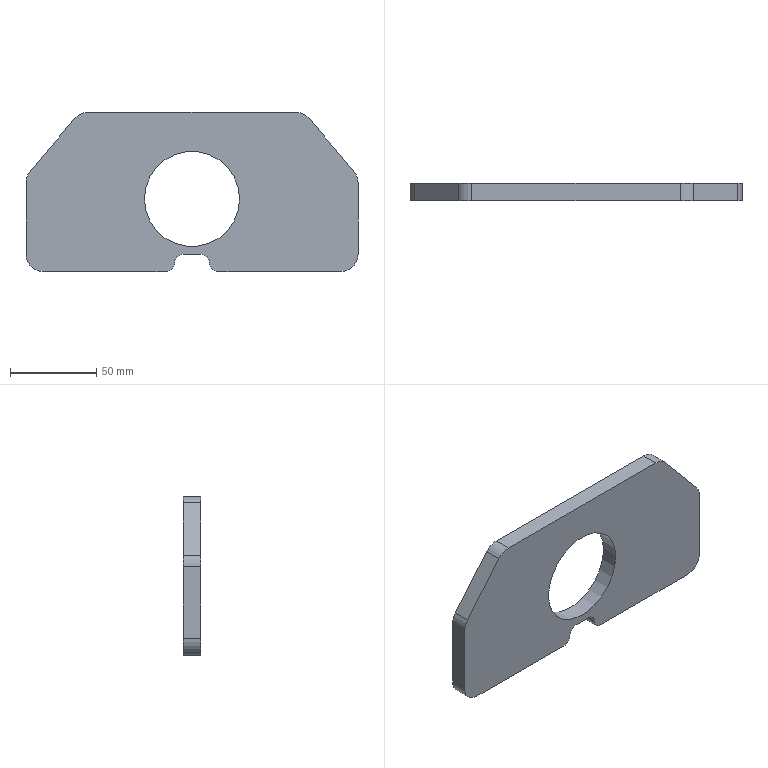Component | SolidWorks | HangingChannelAssembly-2_LiftingLug-3 | 1 solid | 22 faces | box 192 x 10 x 92 mm | volume 138893 mm3 | cylinder 12 | plane 10 | commonest cylinder face diameters 20 x6 10 x4 55 x2 | material Plain Carbon Steel
STEP:
#1=COLOUR_RGB('',0.7922,0.8196,0.9333);
#2=FILL_AREA_STYLE_COLOUR('',#1);
#3=FILL_AREA_STYLE('',(#2));
#4=SURFACE_STYLE_FILL_AREA(#3);
#5=SURFACE_SIDE_STYLE('',(#4));
#6=SURFACE_STYLE_USAGE(.BOTH.,#5);
#7=PRESENTATION_STYLE_ASSIGNMENT((#6));
#8=CARTESIAN_POINT('',(18.377,47.62,81.554));
#9=VERTEX_POINT('',#8);
#10=CARTESIAN_POINT('',(16.212,47.62,81.554));
#11=VERTEX_POINT('',#10);
#12=CARTESIAN_POINT('',(17.295,47.62,81.554));
#13=DIRECTION('',(0.,1.,-0.));
#14=DIRECTION('',(-1.,0.,0.));
#15=AXIS2_PLACEMENT_3D('',#12,#13,#14);
#16=CIRCLE('',#15,1.083);
#17=EDGE_CURVE('',#9,#11,#16,.T.);
#18=ORIENTED_EDGE('',*,*,#17,.T.);
#19=CARTESIAN_POINT('',(16.212,47.226,81.554));
#20=VERTEX_POINT('',#19);
#21=CARTESIAN_POINT('',(16.212,47.62,81.554));
#22=DIRECTION('',(-0.,-1.,0.));
#23=VECTOR('',#22,39.37);
#24=LINE('',#21,#23);
#25=EDGE_CURVE('',#11,#20,#24,.T.);
#26=ORIENTED_EDGE('',*,*,#25,.T.);
#27=CARTESIAN_POINT('',(18.377,47.226,81.554));
#28=VERTEX_POINT('',#27);
#29=CARTESIAN_POINT('',(17.295,47.226,81.554));
#30=DIRECTION('',(0.,1.,-0.));
#31=DIRECTION('',(-1.,0.,0.));
#32=AXIS2_PLACEMENT_3D('',#29,#30,#31);
#33=CIRCLE('',#32,1.083);
#34=EDGE_CURVE('',#28,#20,#33,.T.);
#35=ORIENTED_EDGE('',*,*,#34,.F.);
#36=CARTESIAN_POINT('',(18.377,47.62,81.554));
#37=DIRECTION('',(-0.,-1.,0.));
#38=VECTOR('',#37,39.37);
#39=LINE('',#36,#38);
#40=EDGE_CURVE('',#9,#28,#39,.T.);
#41=ORIENTED_EDGE('',*,*,#40,.F.);
#42=EDGE_LOOP('',(#18,#26,#35,#41));
#43=FACE_OUTER_BOUND('',#42,.T.);
#44=CARTESIAN_POINT('',(17.295,47.62,81.554));
#45=DIRECTION('',(-0.,-1.,0.));
#46=DIRECTION('',(1.,0.,0.));
#47=AXIS2_PLACEMENT_3D('',#44,#45,#46);
#48=CYLINDRICAL_SURFACE('',#47,1.083);
#49=ADVANCED_FACE('',(#43),#48,.F.);
#50=CARTESIAN_POINT('',(16.704,47.62,79.901));
#51=VERTEX_POINT('',#50);
#52=CARTESIAN_POINT('',(13.909,47.62,79.901));
#53=VERTEX_POINT('',#52);
#54=CARTESIAN_POINT('',(21.074,47.62,79.901));
#55=DIRECTION('',(-1.,0.,-0.));
#56=VECTOR('',#55,39.37);
#57=LINE('',#54,#56);
#58=EDGE_CURVE('',#51,#53,#57,.T.);
#59=ORIENTED_EDGE('',*,*,#58,.F.);
#60=CARTESIAN_POINT('',(16.704,47.226,79.901));
#61=VERTEX_POINT('',#60);
#62=CARTESIAN_POINT('',(16.704,47.62,79.901));
#63=DIRECTION('',(-0.,-1.,0.));
#64=VECTOR('',#63,39.37);
#65=LINE('',#62,#64);
#66=EDGE_CURVE('',#51,#61,#65,.T.);
#67=ORIENTED_EDGE('',*,*,#66,.T.);
#68=CARTESIAN_POINT('',(13.909,47.226,79.901));
#69=VERTEX_POINT('',#68);
#70=CARTESIAN_POINT('',(21.074,47.226,79.901));
#71=DIRECTION('',(-1.,0.,-0.));
#72=VECTOR('',#71,39.37);
#73=LINE('',#70,#72);
#74=EDGE_CURVE('',#61,#69,#73,.T.);
#75=ORIENTED_EDGE('',*,*,#74,.T.);
#76=CARTESIAN_POINT('',(13.909,47.62,79.901));
#77=DIRECTION('',(0.,1.,-0.));
#78=VECTOR('',#77,39.37);
#79=LINE('',#76,#78);
#80=EDGE_CURVE('',#69,#53,#79,.T.);
#81=ORIENTED_EDGE('',*,*,#80,.T.);
#82=EDGE_LOOP('',(#59,#67,#75,#81));
#83=FACE_OUTER_BOUND('',#82,.T.);
#84=CARTESIAN_POINT('',(21.074,47.62,79.901));
#85=DIRECTION('',(0.,0.,1.));
#86=DIRECTION('',(0.,1.,-0.));
#87=AXIS2_PLACEMENT_3D('',#84,#85,#86);
#88=PLANE('',#87);
#89=ADVANCED_FACE('',(#83),#88,.F.);
#90=CARTESIAN_POINT('',(17.492,47.62,80.294));
#91=VERTEX_POINT('',#90);
#92=CARTESIAN_POINT('',(17.098,47.62,80.294));
#93=VERTEX_POINT('',#92);
#94=CARTESIAN_POINT('',(16.901,47.62,80.294));
#95=DIRECTION('',(-1.,0.,-0.));
#96=VECTOR('',#95,39.37);
#97=LINE('',#94,#96);
#98=EDGE_CURVE('',#91,#93,#97,.T.);
#99=ORIENTED_EDGE('',*,*,#98,.T.);
#100=CARTESIAN_POINT('',(16.901,47.62,80.098));
#101=VERTEX_POINT('',#100);
#102=CARTESIAN_POINT('',(17.098,47.62,80.098));
#103=DIRECTION('',(-0.,-1.,0.));
#104=DIRECTION('',(-1.,0.,0.));
#105=AXIS2_PLACEMENT_3D('',#102,#103,#104);
#106=CIRCLE('',#105,0.1969);
#107=EDGE_CURVE('',#93,#101,#106,.T.);
#108=ORIENTED_EDGE('',*,*,#107,.T.);
#109=CARTESIAN_POINT('',(16.704,47.62,80.098));
#110=DIRECTION('',(0.,1.,-0.));
#111=DIRECTION('',(-1.,0.,0.));
#112=AXIS2_PLACEMENT_3D('',#109,#110,#111);
#113=CIRCLE('',#112,0.1969);
#114=EDGE_CURVE('',#101,#51,#113,.T.);
#115=ORIENTED_EDGE('',*,*,#114,.T.);
#116=ORIENTED_EDGE('',*,*,#58,.T.);
#117=CARTESIAN_POINT('',(13.515,47.62,80.294));
#118=VERTEX_POINT('',#117);
#119=CARTESIAN_POINT('',(13.909,47.62,80.294));
#120=DIRECTION('',(0.,1.,-0.));
#121=DIRECTION('',(-1.,0.,0.));
#122=AXIS2_PLACEMENT_3D('',#119,#120,#121);
#123=CIRCLE('',#122,0.3937);
#124=EDGE_CURVE('',#53,#118,#123,.T.);
#125=ORIENTED_EDGE('',*,*,#124,.T.);
#126=CARTESIAN_POINT('',(13.515,47.62,81.923));
#127=VERTEX_POINT('',#126);
#128=CARTESIAN_POINT('',(13.515,47.62,79.901));
#129=DIRECTION('',(0.,0.,1.));
#130=VECTOR('',#129,39.37);
#131=LINE('',#128,#130);
#132=EDGE_CURVE('',#118,#127,#131,.T.);
#133=ORIENTED_EDGE('',*,*,#132,.T.);
#134=CARTESIAN_POINT('',(13.607,47.62,82.176));
#135=VERTEX_POINT('',#134);
#136=CARTESIAN_POINT('',(13.909,47.62,81.923));
#137=DIRECTION('',(0.,1.,-0.));
#138=DIRECTION('',(-1.,0.,0.));
#139=AXIS2_PLACEMENT_3D('',#136,#137,#138);
#140=CIRCLE('',#139,0.3937);
#141=EDGE_CURVE('',#127,#135,#140,.T.);
#142=ORIENTED_EDGE('',*,*,#141,.T.);
#143=CARTESIAN_POINT('',(14.618,47.62,83.382));
#144=VERTEX_POINT('',#143);
#145=CARTESIAN_POINT('',(14.736,47.62,83.523));
#146=DIRECTION('',(0.6422,0.,0.7665));
#147=VECTOR('',#146,39.37);
#148=LINE('',#145,#147);
#149=EDGE_CURVE('',#135,#144,#148,.T.);
#150=ORIENTED_EDGE('',*,*,#149,.T.);
#151=CARTESIAN_POINT('',(14.919,47.62,83.523));
#152=VERTEX_POINT('',#151);
#153=CARTESIAN_POINT('',(14.919,47.62,83.129));
#154=DIRECTION('',(0.,1.,-0.));
#155=DIRECTION('',(-1.,0.,0.));
#156=AXIS2_PLACEMENT_3D('',#153,#154,#155);
#157=CIRCLE('',#156,0.3937);
#158=EDGE_CURVE('',#144,#152,#157,.T.);
#159=ORIENTED_EDGE('',*,*,#158,.T.);
#160=CARTESIAN_POINT('',(19.67,47.62,83.523));
#161=VERTEX_POINT('',#160);
#162=CARTESIAN_POINT('',(14.736,47.62,83.523));
#163=DIRECTION('',(1.,-0.,-0.));
#164=VECTOR('',#163,39.37);
#165=LINE('',#162,#164);
#166=EDGE_CURVE('',#152,#161,#165,.T.);
#167=ORIENTED_EDGE('',*,*,#166,.T.);
#168=CARTESIAN_POINT('',(19.972,47.62,83.382));
#169=VERTEX_POINT('',#168);
#170=CARTESIAN_POINT('',(19.67,47.62,83.129));
#171=DIRECTION('',(0.,1.,-0.));
#172=DIRECTION('',(-1.,0.,0.));
#173=AXIS2_PLACEMENT_3D('',#170,#171,#172);
#174=CIRCLE('',#173,0.3937);
#175=EDGE_CURVE('',#161,#169,#174,.T.);
#176=ORIENTED_EDGE('',*,*,#175,.T.);
#177=CARTESIAN_POINT('',(20.982,47.62,82.176));
#178=VERTEX_POINT('',#177);
#179=CARTESIAN_POINT('',(19.854,47.62,83.523));
#180=DIRECTION('',(0.6422,-0.,-0.7665));
#181=VECTOR('',#180,39.37);
#182=LINE('',#179,#181);
#183=EDGE_CURVE('',#169,#178,#182,.T.);
#184=ORIENTED_EDGE('',*,*,#183,.T.);
#185=CARTESIAN_POINT('',(21.074,47.62,81.923));
#186=VERTEX_POINT('',#185);
#187=CARTESIAN_POINT('',(20.681,47.62,81.923));
#188=DIRECTION('',(0.,1.,-0.));
#189=DIRECTION('',(-1.,0.,0.));
#190=AXIS2_PLACEMENT_3D('',#187,#188,#189);
#191=CIRCLE('',#190,0.3937);
#192=EDGE_CURVE('',#178,#186,#191,.T.);
#193=ORIENTED_EDGE('',*,*,#192,.T.);
#194=CARTESIAN_POINT('',(21.074,47.62,80.294));
#195=VERTEX_POINT('',#194);
#196=CARTESIAN_POINT('',(21.074,47.62,79.901));
#197=DIRECTION('',(-0.,-0.,-1.));
#198=VECTOR('',#197,39.37);
#199=LINE('',#196,#198);
#200=EDGE_CURVE('',#186,#195,#199,.T.);
#201=ORIENTED_EDGE('',*,*,#200,.T.);
#202=CARTESIAN_POINT('',(20.681,47.62,79.901));
#203=VERTEX_POINT('',#202);
#204=CARTESIAN_POINT('',(20.681,47.62,80.294));
#205=DIRECTION('',(0.,1.,-0.));
#206=DIRECTION('',(-1.,0.,0.));
#207=AXIS2_PLACEMENT_3D('',#204,#205,#206);
#208=CIRCLE('',#207,0.3937);
#209=EDGE_CURVE('',#195,#203,#208,.T.);
#210=ORIENTED_EDGE('',*,*,#209,.T.);
#211=CARTESIAN_POINT('',(17.885,47.62,79.901));
#212=VERTEX_POINT('',#211);
#213=CARTESIAN_POINT('',(21.074,47.62,79.901));
#214=DIRECTION('',(-1.,0.,-0.));
#215=VECTOR('',#214,39.37);
#216=LINE('',#213,#215);
#217=EDGE_CURVE('',#203,#212,#216,.T.);
#218=ORIENTED_EDGE('',*,*,#217,.T.);
#219=CARTESIAN_POINT('',(17.688,47.62,80.098));
#220=VERTEX_POINT('',#219);
#221=CARTESIAN_POINT('',(17.885,47.62,80.098));
#222=DIRECTION('',(0.,1.,-0.));
#223=DIRECTION('',(-1.,0.,0.));
#224=AXIS2_PLACEMENT_3D('',#221,#222,#223);
#225=CIRCLE('',#224,0.1969);
#226=EDGE_CURVE('',#212,#220,#225,.T.);
#227=ORIENTED_EDGE('',*,*,#226,.T.);
#228=CARTESIAN_POINT('',(17.492,47.62,80.098));
#229=DIRECTION('',(-0.,-1.,0.));
#230=DIRECTION('',(-1.,0.,0.));
#231=AXIS2_PLACEMENT_3D('',#228,#229,#230);
#232=CIRCLE('',#231,0.1969);
#233=EDGE_CURVE('',#220,#91,#232,.T.);
#234=ORIENTED_EDGE('',*,*,#233,.T.);
#235=EDGE_LOOP('',(#99,#108,#115,#116,#125,#133,#142,#150,#159,#167,#176,#184,#193,#201,#210,#218,#227,#234));
#236=FACE_OUTER_BOUND('',#235,.T.);
#237=ORIENTED_EDGE('',*,*,#17,.F.);
#238=CARTESIAN_POINT('',(17.295,47.62,81.554));
#239=DIRECTION('',(0.,1.,-0.));
#240=DIRECTION('',(-1.,0.,0.));
#241=AXIS2_PLACEMENT_3D('',#238,#239,#240);
#242=CIRCLE('',#241,1.083);
#243=EDGE_CURVE('',#11,#9,#242,.T.);
#244=ORIENTED_EDGE('',*,*,#243,.F.);
#245=EDGE_LOOP('',(#237,#244));
#246=FACE_BOUND('',#245,.T.);
#247=CARTESIAN_POINT('',(21.074,47.62,79.901));
#248=DIRECTION('',(0.,1.,-0.));
#249=DIRECTION('',(-1.,0.,-0.));
#250=AXIS2_PLACEMENT_3D('',#247,#248,#249);
#251=PLANE('',#250);
#252=ADVANCED_FACE('',(#236,#246),#251,.T.);
#253=ORIENTED_EDGE('',*,*,#74,.F.);
#254=CARTESIAN_POINT('',(16.901,47.226,80.098));
#255=VERTEX_POINT('',#254);
#256=CARTESIAN_POINT('',(16.704,47.226,80.098));
#257=DIRECTION('',(-0.,-1.,0.));
#258=DIRECTION('',(-1.,0.,0.));
#259=AXIS2_PLACEMENT_3D('',#256,#257,#258);
#260=CIRCLE('',#259,0.1969);
#261=EDGE_CURVE('',#61,#255,#260,.T.);
#262=ORIENTED_EDGE('',*,*,#261,.T.);
#263=CARTESIAN_POINT('',(17.098,47.226,80.294));
#264=VERTEX_POINT('',#263);
#265=CARTESIAN_POINT('',(17.098,47.226,80.098));
#266=DIRECTION('',(0.,1.,-0.));
#267=DIRECTION('',(-1.,0.,0.));
#268=AXIS2_PLACEMENT_3D('',#265,#266,#267);
#269=CIRCLE('',#268,0.1969);
#270=EDGE_CURVE('',#255,#264,#269,.T.);
#271=ORIENTED_EDGE('',*,*,#270,.T.);
#272=CARTESIAN_POINT('',(17.492,47.226,80.294));
#273=VERTEX_POINT('',#272);
#274=CARTESIAN_POINT('',(16.901,47.226,80.294));
#275=DIRECTION('',(-1.,0.,-0.));
#276=VECTOR('',#275,39.37);
#277=LINE('',#274,#276);
#278=EDGE_CURVE('',#273,#264,#277,.T.);
#279=ORIENTED_EDGE('',*,*,#278,.F.);
#280=CARTESIAN_POINT('',(17.688,47.226,80.098));
#281=VERTEX_POINT('',#280);
#282=CARTESIAN_POINT('',(17.492,47.226,80.098));
#283=DIRECTION('',(0.,1.,-0.));
#284=DIRECTION('',(-1.,0.,0.));
#285=AXIS2_PLACEMENT_3D('',#282,#283,#284);
#286=CIRCLE('',#285,0.1969);
#287=EDGE_CURVE('',#273,#281,#286,.T.);
#288=ORIENTED_EDGE('',*,*,#287,.T.);
#289=CARTESIAN_POINT('',(17.885,47.226,79.901));
#290=VERTEX_POINT('',#289);
#291=CARTESIAN_POINT('',(17.885,47.226,80.098));
#292=DIRECTION('',(-0.,-1.,0.));
#293=DIRECTION('',(-1.,0.,0.));
#294=AXIS2_PLACEMENT_3D('',#291,#292,#293);
#295=CIRCLE('',#294,0.1969);
#296=EDGE_CURVE('',#281,#290,#295,.T.);
#297=ORIENTED_EDGE('',*,*,#296,.T.);
#298=CARTESIAN_POINT('',(20.681,47.226,79.901));
#299=VERTEX_POINT('',#298);
#300=CARTESIAN_POINT('',(21.074,47.226,79.901));
#301=DIRECTION('',(-1.,0.,-0.));
#302=VECTOR('',#301,39.37);
#303=LINE('',#300,#302);
#304=EDGE_CURVE('',#299,#290,#303,.T.);
#305=ORIENTED_EDGE('',*,*,#304,.F.);
#306=CARTESIAN_POINT('',(21.074,47.226,80.294));
#307=VERTEX_POINT('',#306);
#308=CARTESIAN_POINT('',(20.681,47.226,80.294));
#309=DIRECTION('',(-0.,-1.,0.));
#310=DIRECTION('',(-1.,0.,0.));
#311=AXIS2_PLACEMENT_3D('',#308,#309,#310);
#312=CIRCLE('',#311,0.3937);
#313=EDGE_CURVE('',#299,#307,#312,.T.);
#314=ORIENTED_EDGE('',*,*,#313,.T.);
#315=CARTESIAN_POINT('',(21.074,47.226,81.923));
#316=VERTEX_POINT('',#315);
#317=CARTESIAN_POINT('',(21.074,47.226,79.901));
#318=DIRECTION('',(-0.,-0.,-1.));
#319=VECTOR('',#318,39.37);
#320=LINE('',#317,#319);
#321=EDGE_CURVE('',#316,#307,#320,.T.);
#322=ORIENTED_EDGE('',*,*,#321,.F.);
#323=CARTESIAN_POINT('',(20.982,47.226,82.176));
#324=VERTEX_POINT('',#323);
#325=CARTESIAN_POINT('',(20.681,47.226,81.923));
#326=DIRECTION('',(-0.,-1.,0.));
#327=DIRECTION('',(-1.,0.,-0.));
#328=AXIS2_PLACEMENT_3D('',#325,#326,#327);
#329=CIRCLE('',#328,0.3937);
#330=EDGE_CURVE('',#316,#324,#329,.T.);
#331=ORIENTED_EDGE('',*,*,#330,.T.);
#332=CARTESIAN_POINT('',(19.972,47.226,83.382));
#333=VERTEX_POINT('',#332);
#334=CARTESIAN_POINT('',(19.854,47.226,83.523));
#335=DIRECTION('',(0.6422,-0.,-0.7665));
#336=VECTOR('',#335,39.37);
#337=LINE('',#334,#336);
#338=EDGE_CURVE('',#333,#324,#337,.T.);
#339=ORIENTED_EDGE('',*,*,#338,.F.);
#340=CARTESIAN_POINT('',(19.67,47.226,83.523));
#341=VERTEX_POINT('',#340);
#342=CARTESIAN_POINT('',(19.67,47.226,83.129));
#343=DIRECTION('',(-0.,-1.,0.));
#344=DIRECTION('',(-1.,0.,0.));
#345=AXIS2_PLACEMENT_3D('',#342,#343,#344);
#346=CIRCLE('',#345,0.3937);
#347=EDGE_CURVE('',#333,#341,#346,.T.);
#348=ORIENTED_EDGE('',*,*,#347,.T.);
#349=CARTESIAN_POINT('',(14.919,47.226,83.523));
#350=VERTEX_POINT('',#349);
#351=CARTESIAN_POINT('',(14.736,47.226,83.523));
#352=DIRECTION('',(1.,-0.,-0.));
#353=VECTOR('',#352,39.37);
#354=LINE('',#351,#353);
#355=EDGE_CURVE('',#350,#341,#354,.T.);
#356=ORIENTED_EDGE('',*,*,#355,.F.);
#357=CARTESIAN_POINT('',(14.618,47.226,83.382));
#358=VERTEX_POINT('',#357);
#359=CARTESIAN_POINT('',(14.919,47.226,83.129));
#360=DIRECTION('',(-0.,-1.,0.));
#361=DIRECTION('',(-1.,0.,0.));
#362=AXIS2_PLACEMENT_3D('',#359,#360,#361);
#363=CIRCLE('',#362,0.3937);
#364=EDGE_CURVE('',#350,#358,#363,.T.);
#365=ORIENTED_EDGE('',*,*,#364,.T.);
#366=CARTESIAN_POINT('',(13.607,47.226,82.176));
#367=VERTEX_POINT('',#366);
#368=CARTESIAN_POINT('',(14.736,47.226,83.523));
#369=DIRECTION('',(0.6422,0.,0.7665));
#370=VECTOR('',#369,39.37);
#371=LINE('',#368,#370);
#372=EDGE_CURVE('',#367,#358,#371,.T.);
#373=ORIENTED_EDGE('',*,*,#372,.F.);
#374=CARTESIAN_POINT('',(13.515,47.226,81.923));
#375=VERTEX_POINT('',#374);
#376=CARTESIAN_POINT('',(13.909,47.226,81.923));
#377=DIRECTION('',(-0.,-1.,0.));
#378=DIRECTION('',(-1.,0.,0.));
#379=AXIS2_PLACEMENT_3D('',#376,#377,#378);
#380=CIRCLE('',#379,0.3937);
#381=EDGE_CURVE('',#367,#375,#380,.T.);
#382=ORIENTED_EDGE('',*,*,#381,.T.);
#383=CARTESIAN_POINT('',(13.515,47.226,80.294));
#384=VERTEX_POINT('',#383);
#385=CARTESIAN_POINT('',(13.515,47.226,79.901));
#386=DIRECTION('',(0.,0.,1.));
#387=VECTOR('',#386,39.37);
#388=LINE('',#385,#387);
#389=EDGE_CURVE('',#384,#375,#388,.T.);
#390=ORIENTED_EDGE('',*,*,#389,.F.);
#391=CARTESIAN_POINT('',(13.909,47.226,80.294));
#392=DIRECTION('',(-0.,-1.,0.));
#393=DIRECTION('',(-1.,0.,0.));
#394=AXIS2_PLACEMENT_3D('',#391,#392,#393);
#395=CIRCLE('',#394,0.3937);
#396=EDGE_CURVE('',#384,#69,#395,.T.);
#397=ORIENTED_EDGE('',*,*,#396,.T.);
#398=EDGE_LOOP('',(#253,#262,#271,#279,#288,#297,#305,#314,#322,#331,#339,#348,#356,#365,#373,#382,#390,#397));
#399=FACE_OUTER_BOUND('',#398,.T.);
#400=ORIENTED_EDGE('',*,*,#34,.T.);
#401=CARTESIAN_POINT('',(17.295,47.226,81.554));
#402=DIRECTION('',(0.,1.,-0.));
#403=DIRECTION('',(-1.,0.,0.));
#404=AXIS2_PLACEMENT_3D('',#401,#402,#403);
#405=CIRCLE('',#404,1.083);
#406=EDGE_CURVE('',#20,#28,#405,.T.);
#407=ORIENTED_EDGE('',*,*,#406,.T.);
#408=EDGE_LOOP('',(#400,#407));
#409=FACE_BOUND('',#408,.T.);
#410=CARTESIAN_POINT('',(21.074,47.226,79.901));
#411=DIRECTION('',(0.,1.,-0.));
#412=DIRECTION('',(-1.,0.,-0.));
#413=AXIS2_PLACEMENT_3D('',#410,#411,#412);
#414=PLANE('',#413);
#415=ADVANCED_FACE('',(#399,#409),#414,.F.);
#416=ORIENTED_EDGE('',*,*,#200,.F.);
#417=CARTESIAN_POINT('',(21.074,47.62,81.923));
#418=DIRECTION('',(-0.,-1.,0.));
#419=VECTOR('',#418,39.37);
#420=LINE('',#417,#419);
#421=EDGE_CURVE('',#186,#316,#420,.T.);
#422=ORIENTED_EDGE('',*,*,#421,.T.);
#423=ORIENTED_EDGE('',*,*,#321,.T.);
#424=CARTESIAN_POINT('',(21.074,47.62,80.294));
#425=DIRECTION('',(0.,1.,-0.));
#426=VECTOR('',#425,39.37);
#427=LINE('',#424,#426);
#428=EDGE_CURVE('',#307,#195,#427,.T.);
#429=ORIENTED_EDGE('',*,*,#428,.T.);
#430=EDGE_LOOP('',(#416,#422,#423,#429));
#431=FACE_OUTER_BOUND('',#430,.T.);
#432=CARTESIAN_POINT('',(21.074,47.62,79.901));
#433=DIRECTION('',(-1.,0.,0.));
#434=DIRECTION('',(-0.,-1.,0.));
#435=AXIS2_PLACEMENT_3D('',#432,#433,#434);
#436=PLANE('',#435);
#437=ADVANCED_FACE('',(#431),#436,.F.);
#438=ORIENTED_EDGE('',*,*,#304,.T.);
#439=CARTESIAN_POINT('',(17.885,47.62,79.901));
#440=DIRECTION('',(0.,1.,-0.));
#441=VECTOR('',#440,39.37);
#442=LINE('',#439,#441);
#443=EDGE_CURVE('',#290,#212,#442,.T.);
#444=ORIENTED_EDGE('',*,*,#443,.T.);
#445=ORIENTED_EDGE('',*,*,#217,.F.);
#446=CARTESIAN_POINT('',(20.681,47.62,79.901));
#447=DIRECTION('',(-0.,-1.,0.));
#448=VECTOR('',#447,39.37);
#449=LINE('',#446,#448);
#450=EDGE_CURVE('',#203,#299,#449,.T.);
#451=ORIENTED_EDGE('',*,*,#450,.T.);
#452=EDGE_LOOP('',(#438,#444,#445,#451));
#453=FACE_OUTER_BOUND('',#452,.T.);
#454=CARTESIAN_POINT('',(21.074,47.62,79.901));
#455=DIRECTION('',(0.,0.,1.));
#456=DIRECTION('',(0.,1.,-0.));
#457=AXIS2_PLACEMENT_3D('',#454,#455,#456);
#458=PLANE('',#457);
#459=ADVANCED_FACE('',(#453),#458,.F.);
#460=ORIENTED_EDGE('',*,*,#389,.T.);
#461=CARTESIAN_POINT('',(13.515,47.62,81.923));
#462=DIRECTION('',(0.,1.,-0.));
#463=VECTOR('',#462,39.37);
#464=LINE('',#461,#463);
#465=EDGE_CURVE('',#375,#127,#464,.T.);
#466=ORIENTED_EDGE('',*,*,#465,.T.);
#467=ORIENTED_EDGE('',*,*,#132,.F.);
#468=CARTESIAN_POINT('',(13.515,47.62,80.294));
#469=DIRECTION('',(-0.,-1.,0.));
#470=VECTOR('',#469,39.37);
#471=LINE('',#468,#470);
#472=EDGE_CURVE('',#118,#384,#471,.T.);
#473=ORIENTED_EDGE('',*,*,#472,.T.);
#474=EDGE_LOOP('',(#460,#466,#467,#473));
#475=FACE_OUTER_BOUND('',#474,.T.);
#476=CARTESIAN_POINT('',(13.515,47.62,79.901));
#477=DIRECTION('',(1.,-0.,-0.));
#478=DIRECTION('',(0.,1.,-0.));
#479=AXIS2_PLACEMENT_3D('',#476,#477,#478);
#480=PLANE('',#479);
#481=ADVANCED_FACE('',(#475),#480,.F.);
#482=ORIENTED_EDGE('',*,*,#372,.T.);
#483=CARTESIAN_POINT('',(14.618,47.62,83.382));
#484=DIRECTION('',(0.,1.,-0.));
#485=VECTOR('',#484,39.37);
#486=LINE('',#483,#485);
#487=EDGE_CURVE('',#358,#144,#486,.T.);
#488=ORIENTED_EDGE('',*,*,#487,.T.);
#489=ORIENTED_EDGE('',*,*,#149,.F.);
#490=CARTESIAN_POINT('',(13.607,47.62,82.176));
#491=DIRECTION('',(-0.,-1.,0.));
#492=VECTOR('',#491,39.37);
#493=LINE('',#490,#492);
#494=EDGE_CURVE('',#135,#367,#493,.T.);
#495=ORIENTED_EDGE('',*,*,#494,.T.);
#496=EDGE_LOOP('',(#482,#488,#489,#495));
#497=FACE_OUTER_BOUND('',#496,.T.);
#498=CARTESIAN_POINT('',(14.736,47.62,83.523));
#499=DIRECTION('',(0.7665,-0.,-0.6422));
#500=DIRECTION('',(-0.6422,-0.,-0.7665));
#501=AXIS2_PLACEMENT_3D('',#498,#499,#500);
#502=PLANE('',#501);
#503=ADVANCED_FACE('',(#497),#502,.F.);
#504=ORIENTED_EDGE('',*,*,#355,.T.);
#505=CARTESIAN_POINT('',(19.67,47.62,83.523));
#506=DIRECTION('',(0.,1.,-0.));
#507=VECTOR('',#506,39.37);
#508=LINE('',#505,#507);
#509=EDGE_CURVE('',#341,#161,#508,.T.);
#510=ORIENTED_EDGE('',*,*,#509,.T.);
#511=ORIENTED_EDGE('',*,*,#166,.F.);
#512=CARTESIAN_POINT('',(14.919,47.62,83.523));
#513=DIRECTION('',(-0.,-1.,0.));
#514=VECTOR('',#513,39.37);
#515=LINE('',#512,#514);
#516=EDGE_CURVE('',#152,#350,#515,.T.);
#517=ORIENTED_EDGE('',*,*,#516,.T.);
#518=EDGE_LOOP('',(#504,#510,#511,#517));
#519=FACE_OUTER_BOUND('',#518,.T.);
#520=CARTESIAN_POINT('',(14.736,47.62,83.523));
#521=DIRECTION('',(-0.,-0.,-1.));
#522=DIRECTION('',(-1.,0.,0.));
#523=AXIS2_PLACEMENT_3D('',#520,#521,#522);
#524=PLANE('',#523);
#525=ADVANCED_FACE('',(#519),#524,.F.);
#526=ORIENTED_EDGE('',*,*,#338,.T.);
#527=CARTESIAN_POINT('',(20.982,47.62,82.176));
#528=DIRECTION('',(0.,1.,-0.));
#529=VECTOR('',#528,39.37);
#530=LINE('',#527,#529);
#531=EDGE_CURVE('',#324,#178,#530,.T.);
#532=ORIENTED_EDGE('',*,*,#531,.T.);
#533=ORIENTED_EDGE('',*,*,#183,.F.);
#534=CARTESIAN_POINT('',(19.972,47.62,83.382));
#535=DIRECTION('',(-0.,-1.,0.));
#536=VECTOR('',#535,39.37);
#537=LINE('',#534,#536);
#538=EDGE_CURVE('',#169,#333,#537,.T.);
#539=ORIENTED_EDGE('',*,*,#538,.T.);
#540=EDGE_LOOP('',(#526,#532,#533,#539));
#541=FACE_OUTER_BOUND('',#540,.T.);
#542=CARTESIAN_POINT('',(19.854,47.62,83.523));
#543=DIRECTION('',(-0.7665,-0.,-0.6422));
#544=DIRECTION('',(-0.6422,0.,0.7665));
#545=AXIS2_PLACEMENT_3D('',#542,#543,#544);
#546=PLANE('',#545);
#547=ADVANCED_FACE('',(#541),#546,.F.);
#548=ORIENTED_EDGE('',*,*,#25,.F.);
#549=ORIENTED_EDGE('',*,*,#243,.T.);
#550=ORIENTED_EDGE('',*,*,#40,.T.);
#551=ORIENTED_EDGE('',*,*,#406,.F.);
#552=EDGE_LOOP('',(#548,#549,#550,#551));
#553=FACE_OUTER_BOUND('',#552,.T.);
#554=CARTESIAN_POINT('',(17.295,47.62,81.554));
#555=DIRECTION('',(-0.,-1.,0.));
#556=DIRECTION('',(1.,0.,0.));
#557=AXIS2_PLACEMENT_3D('',#554,#555,#556);
#558=CYLINDRICAL_SURFACE('',#557,1.083);
#559=ADVANCED_FACE('',(#553),#558,.F.);
#560=ORIENTED_EDGE('',*,*,#124,.F.);
#561=ORIENTED_EDGE('',*,*,#80,.F.);
#562=ORIENTED_EDGE('',*,*,#396,.F.);
#563=ORIENTED_EDGE('',*,*,#472,.F.);
#564=EDGE_LOOP('',(#560,#561,#562,#563));
#565=FACE_OUTER_BOUND('',#564,.T.);
#566=CARTESIAN_POINT('',(13.909,47.62,80.294));
#567=DIRECTION('',(-0.,-1.,0.));
#568=DIRECTION('',(1.,0.,0.));
#569=AXIS2_PLACEMENT_3D('',#566,#567,#568);
#570=CYLINDRICAL_SURFACE('',#569,0.3937);
#571=ADVANCED_FACE('',(#565),#570,.T.);
#572=ORIENTED_EDGE('',*,*,#209,.F.);
#573=ORIENTED_EDGE('',*,*,#428,.F.);
#574=ORIENTED_EDGE('',*,*,#313,.F.);
#575=ORIENTED_EDGE('',*,*,#450,.F.);
#576=EDGE_LOOP('',(#572,#573,#574,#575));
#577=FACE_OUTER_BOUND('',#576,.T.);
#578=CARTESIAN_POINT('',(20.681,47.62,80.294));
#579=DIRECTION('',(-0.,-1.,0.));
#580=DIRECTION('',(1.,0.,0.));
#581=AXIS2_PLACEMENT_3D('',#578,#579,#580);
#582=CYLINDRICAL_SURFACE('',#581,0.3937);
#583=ADVANCED_FACE('',(#577),#582,.T.);
#584=ORIENTED_EDGE('',*,*,#192,.F.);
#585=ORIENTED_EDGE('',*,*,#531,.F.);
#586=ORIENTED_EDGE('',*,*,#330,.F.);
#587=ORIENTED_EDGE('',*,*,#421,.F.);
#588=EDGE_LOOP('',(#584,#585,#586,#587));
#589=FACE_OUTER_BOUND('',#588,.T.);
#590=CARTESIAN_POINT('',(20.681,47.62,81.923));
#591=DIRECTION('',(-0.,-1.,0.));
#592=DIRECTION('',(1.,0.,0.));
#593=AXIS2_PLACEMENT_3D('',#590,#591,#592);
#594=CYLINDRICAL_SURFACE('',#593,0.3937);
#595=ADVANCED_FACE('',(#589),#594,.T.);
#596=ORIENTED_EDGE('',*,*,#175,.F.);
#597=ORIENTED_EDGE('',*,*,#509,.F.);
#598=ORIENTED_EDGE('',*,*,#347,.F.);
#599=ORIENTED_EDGE('',*,*,#538,.F.);
#600=EDGE_LOOP('',(#596,#597,#598,#599));
#601=FACE_OUTER_BOUND('',#600,.T.);
#602=CARTESIAN_POINT('',(19.67,47.62,83.129));
#603=DIRECTION('',(-0.,-1.,0.));
#604=DIRECTION('',(1.,0.,0.));
#605=AXIS2_PLACEMENT_3D('',#602,#603,#604);
#606=CYLINDRICAL_SURFACE('',#605,0.3937);
#607=ADVANCED_FACE('',(#601),#606,.T.);
#608=ORIENTED_EDGE('',*,*,#158,.F.);
#609=ORIENTED_EDGE('',*,*,#487,.F.);
#610=ORIENTED_EDGE('',*,*,#364,.F.);
#611=ORIENTED_EDGE('',*,*,#516,.F.);
#612=EDGE_LOOP('',(#608,#609,#610,#611));
#613=FACE_OUTER_BOUND('',#612,.T.);
#614=CARTESIAN_POINT('',(14.919,47.62,83.129));
#615=DIRECTION('',(-0.,-1.,0.));
#616=DIRECTION('',(1.,0.,0.));
#617=AXIS2_PLACEMENT_3D('',#614,#615,#616);
#618=CYLINDRICAL_SURFACE('',#617,0.3937);
#619=ADVANCED_FACE('',(#613),#618,.T.);
#620=ORIENTED_EDGE('',*,*,#141,.F.);
#621=ORIENTED_EDGE('',*,*,#465,.F.);
#622=ORIENTED_EDGE('',*,*,#381,.F.);
#623=ORIENTED_EDGE('',*,*,#494,.F.);
#624=EDGE_LOOP('',(#620,#621,#622,#623));
#625=FACE_OUTER_BOUND('',#624,.T.);
#626=CARTESIAN_POINT('',(13.909,47.62,81.923));
#627=DIRECTION('',(-0.,-1.,0.));
#628=DIRECTION('',(1.,0.,0.));
#629=AXIS2_PLACEMENT_3D('',#626,#627,#628);
#630=CYLINDRICAL_SURFACE('',#629,0.3937);
#631=ADVANCED_FACE('',(#625),#630,.T.);
#632=ORIENTED_EDGE('',*,*,#98,.F.);
#633=CARTESIAN_POINT('',(17.492,47.226,80.294));
#634=DIRECTION('',(-0.,-1.,0.));
#635=VECTOR('',#634,39.37);
#636=LINE('',#633,#635);
#637=EDGE_CURVE('',#91,#273,#636,.T.);
#638=ORIENTED_EDGE('',*,*,#637,.T.);
#639=ORIENTED_EDGE('',*,*,#278,.T.);
#640=CARTESIAN_POINT('',(17.098,47.62,80.294));
#641=DIRECTION('',(0.,1.,-0.));
#642=VECTOR('',#641,39.37);
#643=LINE('',#640,#642);
#644=EDGE_CURVE('',#264,#93,#643,.T.);
#645=ORIENTED_EDGE('',*,*,#644,.T.);
#646=EDGE_LOOP('',(#632,#638,#639,#645));
#647=FACE_OUTER_BOUND('',#646,.T.);
#648=CARTESIAN_POINT('',(16.901,47.62,80.294));
#649=DIRECTION('',(0.,0.,1.));
#650=DIRECTION('',(0.,1.,-0.));
#651=AXIS2_PLACEMENT_3D('',#648,#649,#650);
#652=PLANE('',#651);
#653=ADVANCED_FACE('',(#647),#652,.F.);
#654=CARTESIAN_POINT('',(16.901,47.226,80.098));
#655=DIRECTION('',(-0.,-1.,0.));
#656=VECTOR('',#655,39.37);
#657=LINE('',#654,#656);
#658=EDGE_CURVE('',#101,#255,#657,.T.);
#659=ORIENTED_EDGE('',*,*,#658,.F.);
#660=ORIENTED_EDGE('',*,*,#107,.F.);
#661=ORIENTED_EDGE('',*,*,#644,.F.);
#662=ORIENTED_EDGE('',*,*,#270,.F.);
#663=EDGE_LOOP('',(#659,#660,#661,#662));
#664=FACE_OUTER_BOUND('',#663,.T.);
#665=CARTESIAN_POINT('',(17.098,47.62,80.098));
#666=DIRECTION('',(0.,1.,-0.));
#667=DIRECTION('',(-1.,0.,0.));
#668=AXIS2_PLACEMENT_3D('',#665,#666,#667);
#669=CYLINDRICAL_SURFACE('',#668,0.1969);
#670=ADVANCED_FACE('',(#664),#669,.F.);
#671=ORIENTED_EDGE('',*,*,#114,.F.);
#672=ORIENTED_EDGE('',*,*,#658,.T.);
#673=ORIENTED_EDGE('',*,*,#261,.F.);
#674=ORIENTED_EDGE('',*,*,#66,.F.);
#675=EDGE_LOOP('',(#671,#672,#673,#674));
#676=FACE_OUTER_BOUND('',#675,.T.);
#677=CARTESIAN_POINT('',(16.704,47.62,80.098));
#678=DIRECTION('',(-0.,-1.,0.));
#679=DIRECTION('',(1.,0.,0.));
#680=AXIS2_PLACEMENT_3D('',#677,#678,#679);
#681=CYLINDRICAL_SURFACE('',#680,0.1969);
#682=ADVANCED_FACE('',(#676),#681,.T.);
#683=ORIENTED_EDGE('',*,*,#637,.F.);
#684=ORIENTED_EDGE('',*,*,#233,.F.);
#685=CARTESIAN_POINT('',(17.688,47.62,80.098));
#686=DIRECTION('',(0.,1.,-0.));
#687=VECTOR('',#686,39.37);
#688=LINE('',#685,#687);
#689=EDGE_CURVE('',#281,#220,#688,.T.);
#690=ORIENTED_EDGE('',*,*,#689,.F.);
#691=ORIENTED_EDGE('',*,*,#287,.F.);
#692=EDGE_LOOP('',(#683,#684,#690,#691));
#693=FACE_OUTER_BOUND('',#692,.T.);
#694=CARTESIAN_POINT('',(17.492,47.62,80.098));
#695=DIRECTION('',(0.,1.,-0.));
#696=DIRECTION('',(-1.,0.,0.));
#697=AXIS2_PLACEMENT_3D('',#694,#695,#696);
#698=CYLINDRICAL_SURFACE('',#697,0.1969);
#699=ADVANCED_FACE('',(#693),#698,.F.);
#700=ORIENTED_EDGE('',*,*,#226,.F.);
#701=ORIENTED_EDGE('',*,*,#443,.F.);
#702=ORIENTED_EDGE('',*,*,#296,.F.);
#703=ORIENTED_EDGE('',*,*,#689,.T.);
#704=EDGE_LOOP('',(#700,#701,#702,#703));
#705=FACE_OUTER_BOUND('',#704,.T.);
#706=CARTESIAN_POINT('',(17.885,47.62,80.098));
#707=DIRECTION('',(-0.,-1.,0.));
#708=DIRECTION('',(1.,0.,0.));
#709=AXIS2_PLACEMENT_3D('',#706,#707,#708);
#710=CYLINDRICAL_SURFACE('',#709,0.1969);
#711=ADVANCED_FACE('',(#705),#710,.T.);
#712=CLOSED_SHELL('',(#49,#89,#252,#415,#437,#459,#481,#503,#525,#547,#559,#571,#583,#595,#607,#619,#631,#653,#670,#682,#699,#711));
#713=MANIFOLD_SOLID_BREP('',#712);
#714=STYLED_ITEM('',(#7),#713);
#715=PRESENTATION_LAYER_ASSIGNMENT('','',(#714));
#716=CARTESIAN_POINT('',(0.,0.,0.));
#717=DIRECTION('',(0.,0.,1.));
#718=DIRECTION('',(1.,0.,0.));
#719=AXIS2_PLACEMENT_3D('',#716,#717,#718);
#720=(LENGTH_UNIT()NAMED_UNIT(*)SI_UNIT($,.METRE.));
#721=LENGTH_MEASURE_WITH_UNIT(LENGTH_MEASURE(0.0254),#720);
#722=DIMENSIONAL_EXPONENTS(1.,0.,0.,0.,0.,0.,0.);
#723=(CONVERSION_BASED_UNIT('',#721)LENGTH_UNIT()NAMED_UNIT(#722));
#724=UNCERTAINTY_MEASURE_WITH_UNIT(LENGTH_MEASURE(0.00001),#723,'','');
#725=(NAMED_UNIT(*)PLANE_ANGLE_UNIT()SI_UNIT($,.RADIAN.));
#726=(NAMED_UNIT(*)SI_UNIT($,.STERADIAN.)SOLID_ANGLE_UNIT());
#727=(GEOMETRIC_REPRESENTATION_CONTEXT(3)GLOBAL_UNCERTAINTY_ASSIGNED_CONTEXT((#724))GLOBAL_UNIT_ASSIGNED_CONTEXT((#723,#725,#726))REPRESENTATION_CONTEXT('',''));
#728=ADVANCED_BREP_SHAPE_REPRESENTATION('',(#713,#719),#727);
#729=(LENGTH_UNIT()NAMED_UNIT(*)SI_UNIT($,.METRE.));
#730=LENGTH_MEASURE_WITH_UNIT(LENGTH_MEASURE(0.0254),#729);
#731=DIMENSIONAL_EXPONENTS(1.,0.,0.,0.,0.,0.,0.);
#732=(CONVERSION_BASED_UNIT('',#730)LENGTH_UNIT()NAMED_UNIT(#731));
#733=UNCERTAINTY_MEASURE_WITH_UNIT(LENGTH_MEASURE(0.00001),#732,'','');
#734=(NAMED_UNIT(*)PLANE_ANGLE_UNIT()SI_UNIT($,.RADIAN.));
#735=(NAMED_UNIT(*)SI_UNIT($,.STERADIAN.)SOLID_ANGLE_UNIT());
#736=(GEOMETRIC_REPRESENTATION_CONTEXT(3)GLOBAL_UNCERTAINTY_ASSIGNED_CONTEXT((#733))GLOBAL_UNIT_ASSIGNED_CONTEXT((#732,#734,#735))REPRESENTATION_CONTEXT('',''));
#737=MECHANICAL_DESIGN_GEOMETRIC_PRESENTATION_REPRESENTATION('',(#714),#736);